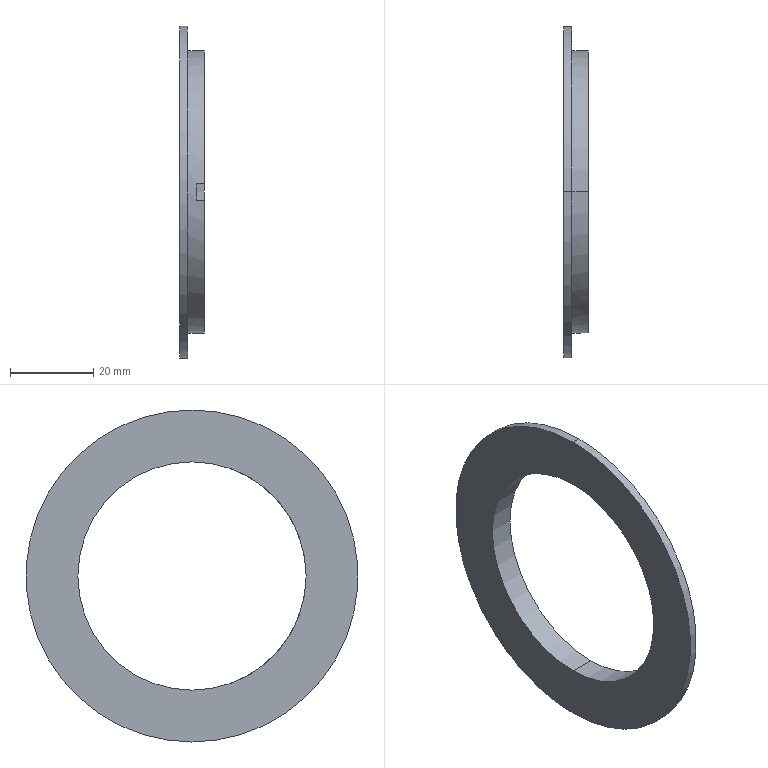Component | SolidWorks | 2InsulatingRing-1 | 1 solid | 12 faces | box 6 x 80 x 80 mm | volume 10273 mm3 | cylinder 6 | plane 6 | commonest cylinder face diameters 55 x2 68 x2 80 x2
build123d program:
from build123d import *

# Parameters (mm, degrees)
SKETCH15_R          = 40
BOSS_EXTRUDE4_DEPTH = 2
SKETCH16_R          = 34
BOSS_EXTRUDE5_DEPTH = 4
SKETCH17_R          = 27.5
CUT_EXTRUDE7_DEPTH  = 34
SKETCH18_W          = 9.008
SKETCH18_H          = 4
CUT_EXTRUDE8_DEPTH  = 57.886


with BuildPart() as part:
    # Sketch15 → Boss-Extrude4 (new body)
    with BuildSketch(Plane(origin=(0, 0, 0), x_dir=(0, 0, -1), z_dir=(1, 0, 0))):
        Circle(SKETCH15_R)
    extrude(amount=BOSS_EXTRUDE4_DEPTH)

    # Sketch16 → Boss-Extrude5 (add)
    with BuildSketch(Plane(origin=(2, 0, 0), x_dir=(0, 0, -1), z_dir=(1, 0, 0))):
        Circle(SKETCH16_R)
    extrude(amount=BOSS_EXTRUDE5_DEPTH)

    # Sketch17 → Cut-Extrude7 (cut)
    with BuildSketch(Plane(origin=(6, 0, 0), x_dir=(0, 0, -1), z_dir=(1, 0, 0))):
        Circle(SKETCH17_R)
    extrude(amount=-CUT_EXTRUDE7_DEPTH, mode=Mode.SUBTRACT)

    # Sketch18 → Cut-Extrude8 (cut, through all)
    with BuildSketch(Plane(origin=(0, 0, 0), x_dir=(1, 0, 0), z_dir=(0, 1, 0))):
        with Locations((8.504, 0)):
            Rectangle(SKETCH18_W, SKETCH18_H)
    extrude(amount=-CUT_EXTRUDE8_DEPTH, mode=Mode.SUBTRACT)


solid = part.part

# Placed as in the assembly
solid = solid.moved(Location((46.957, 1.776, 250), (0, 0, 0)))
STEP:
#1=COLOUR_RGB('',0.7922,0.8196,0.9333);
#2=FILL_AREA_STYLE_COLOUR('',#1);
#3=FILL_AREA_STYLE('',(#2));
#4=SURFACE_STYLE_FILL_AREA(#3);
#5=SURFACE_SIDE_STYLE('',(#4));
#6=SURFACE_STYLE_USAGE(.BOTH.,#5);
#7=PRESENTATION_STYLE_ASSIGNMENT((#6));
#8=CARTESIAN_POINT('',(1.849,0.06992,10.925));
#9=VERTEX_POINT('',#8);
#10=CARTESIAN_POINT('',(1.849,0.06992,8.76));
#11=VERTEX_POINT('',#10);
#12=CARTESIAN_POINT('',(1.849,0.06992,9.843));
#13=DIRECTION('',(1.,0.,0.));
#14=DIRECTION('',(0.,0.,-1.));
#15=AXIS2_PLACEMENT_3D('',#12,#13,#14);
#16=CIRCLE('',#15,1.083);
#17=EDGE_CURVE('',#9,#11,#16,.T.);
#18=ORIENTED_EDGE('',*,*,#17,.F.);
#19=CARTESIAN_POINT('',(2.085,0.06992,10.925));
#20=VERTEX_POINT('',#19);
#21=CARTESIAN_POINT('',(0.7463,0.06992,10.925));
#22=DIRECTION('',(1.,0.,0.));
#23=VECTOR('',#22,39.37);
#24=LINE('',#21,#23);
#25=EDGE_CURVE('',#9,#20,#24,.T.);
#26=ORIENTED_EDGE('',*,*,#25,.T.);
#27=CARTESIAN_POINT('',(2.085,-1.01,9.921));
#28=VERTEX_POINT('',#27);
#29=CARTESIAN_POINT('',(2.085,0.06992,9.843));
#30=DIRECTION('',(1.,0.,0.));
#31=DIRECTION('',(0.,0.,-1.));
#32=AXIS2_PLACEMENT_3D('',#29,#30,#31);
#33=CIRCLE('',#32,1.083);
#34=EDGE_CURVE('',#20,#28,#33,.T.);
#35=ORIENTED_EDGE('',*,*,#34,.T.);
#36=CARTESIAN_POINT('',(2.006,-1.01,9.921));
#37=VERTEX_POINT('',#36);
#38=CARTESIAN_POINT('',(0.7463,-1.01,9.921));
#39=DIRECTION('',(-1.,0.,0.));
#40=VECTOR('',#39,39.37);
#41=LINE('',#38,#40);
#42=EDGE_CURVE('',#28,#37,#41,.T.);
#43=ORIENTED_EDGE('',*,*,#42,.T.);
#44=CARTESIAN_POINT('',(2.006,-1.01,9.764));
#45=VERTEX_POINT('',#44);
#46=CARTESIAN_POINT('',(2.006,0.06992,9.843));
#47=DIRECTION('',(1.,0.,0.));
#48=DIRECTION('',(0.,0.,1.));
#49=AXIS2_PLACEMENT_3D('',#46,#47,#48);
#50=CIRCLE('',#49,1.083);
#51=EDGE_CURVE('',#37,#45,#50,.T.);
#52=ORIENTED_EDGE('',*,*,#51,.T.);
#53=CARTESIAN_POINT('',(2.085,-1.01,9.764));
#54=VERTEX_POINT('',#53);
#55=CARTESIAN_POINT('',(0.7463,-1.01,9.764));
#56=DIRECTION('',(1.,0.,0.));
#57=VECTOR('',#56,39.37);
#58=LINE('',#55,#57);
#59=EDGE_CURVE('',#45,#54,#58,.T.);
#60=ORIENTED_EDGE('',*,*,#59,.T.);
#61=CARTESIAN_POINT('',(2.085,0.06992,8.76));
#62=VERTEX_POINT('',#61);
#63=CARTESIAN_POINT('',(2.085,0.06992,9.843));
#64=DIRECTION('',(1.,0.,0.));
#65=DIRECTION('',(0.,0.,-1.));
#66=AXIS2_PLACEMENT_3D('',#63,#64,#65);
#67=CIRCLE('',#66,1.083);
#68=EDGE_CURVE('',#54,#62,#67,.T.);
#69=ORIENTED_EDGE('',*,*,#68,.T.);
#70=CARTESIAN_POINT('',(0.7463,0.06992,8.76));
#71=DIRECTION('',(1.,0.,0.));
#72=VECTOR('',#71,39.37);
#73=LINE('',#70,#72);
#74=EDGE_CURVE('',#11,#62,#73,.T.);
#75=ORIENTED_EDGE('',*,*,#74,.F.);
#76=EDGE_LOOP('',(#18,#26,#35,#43,#52,#60,#69,#75));
#77=FACE_OUTER_BOUND('',#76,.T.);
#78=CARTESIAN_POINT('',(0.7463,0.06992,9.843));
#79=DIRECTION('',(1.,0.,0.));
#80=DIRECTION('',(0.,0.,-1.));
#81=AXIS2_PLACEMENT_3D('',#78,#79,#80);
#82=CYLINDRICAL_SURFACE('',#81,1.083);
#83=ADVANCED_FACE('',(#77),#82,.F.);
#84=CARTESIAN_POINT('',(2.085,0.06992,8.504));
#85=VERTEX_POINT('',#84);
#86=CARTESIAN_POINT('',(2.085,0.06992,11.181));
#87=VERTEX_POINT('',#86);
#88=CARTESIAN_POINT('',(2.085,0.06992,9.843));
#89=DIRECTION('',(1.,0.,0.));
#90=DIRECTION('',(0.,0.,-1.));
#91=AXIS2_PLACEMENT_3D('',#88,#89,#90);
#92=CIRCLE('',#91,1.339);
#93=EDGE_CURVE('',#85,#87,#92,.T.);
#94=ORIENTED_EDGE('',*,*,#93,.F.);
#95=CARTESIAN_POINT('',(1.927,0.06992,8.504));
#96=VERTEX_POINT('',#95);
#97=CARTESIAN_POINT('',(2.085,0.06992,8.504));
#98=DIRECTION('',(-1.,0.,0.));
#99=VECTOR('',#98,39.37);
#100=LINE('',#97,#99);
#101=EDGE_CURVE('',#85,#96,#100,.T.);
#102=ORIENTED_EDGE('',*,*,#101,.T.);
#103=CARTESIAN_POINT('',(1.927,0.06992,11.181));
#104=VERTEX_POINT('',#103);
#105=CARTESIAN_POINT('',(1.927,0.06992,9.843));
#106=DIRECTION('',(1.,0.,0.));
#107=DIRECTION('',(0.,0.,-1.));
#108=AXIS2_PLACEMENT_3D('',#105,#106,#107);
#109=CIRCLE('',#108,1.339);
#110=EDGE_CURVE('',#96,#104,#109,.T.);
#111=ORIENTED_EDGE('',*,*,#110,.T.);
#112=CARTESIAN_POINT('',(2.085,0.06992,11.181));
#113=DIRECTION('',(-1.,0.,0.));
#114=VECTOR('',#113,39.37);
#115=LINE('',#112,#114);
#116=EDGE_CURVE('',#87,#104,#115,.T.);
#117=ORIENTED_EDGE('',*,*,#116,.F.);
#118=EDGE_LOOP('',(#94,#102,#111,#117));
#119=FACE_OUTER_BOUND('',#118,.T.);
#120=CARTESIAN_POINT('',(2.085,0.06992,9.843));
#121=DIRECTION('',(-1.,0.,0.));
#122=DIRECTION('',(0.,0.,1.));
#123=AXIS2_PLACEMENT_3D('',#120,#121,#122);
#124=CYLINDRICAL_SURFACE('',#123,1.339);
#125=ADVANCED_FACE('',(#119),#124,.T.);
#126=CARTESIAN_POINT('',(1.927,0.06992,8.268));
#127=VERTEX_POINT('',#126);
#128=CARTESIAN_POINT('',(1.927,0.06992,11.417));
#129=VERTEX_POINT('',#128);
#130=CARTESIAN_POINT('',(1.927,0.06992,9.843));
#131=DIRECTION('',(1.,0.,0.));
#132=DIRECTION('',(0.,0.,-1.));
#133=AXIS2_PLACEMENT_3D('',#130,#131,#132);
#134=CIRCLE('',#133,1.575);
#135=EDGE_CURVE('',#127,#129,#134,.T.);
#136=ORIENTED_EDGE('',*,*,#135,.F.);
#137=CARTESIAN_POINT('',(1.849,0.06992,8.268));
#138=VERTEX_POINT('',#137);
#139=CARTESIAN_POINT('',(1.927,0.06992,8.268));
#140=DIRECTION('',(-1.,0.,0.));
#141=VECTOR('',#140,39.37);
#142=LINE('',#139,#141);
#143=EDGE_CURVE('',#127,#138,#142,.T.);
#144=ORIENTED_EDGE('',*,*,#143,.T.);
#145=CARTESIAN_POINT('',(1.849,0.06992,11.417));
#146=VERTEX_POINT('',#145);
#147=CARTESIAN_POINT('',(1.849,0.06992,9.843));
#148=DIRECTION('',(1.,0.,0.));
#149=DIRECTION('',(0.,0.,-1.));
#150=AXIS2_PLACEMENT_3D('',#147,#148,#149);
#151=CIRCLE('',#150,1.575);
#152=EDGE_CURVE('',#138,#146,#151,.T.);
#153=ORIENTED_EDGE('',*,*,#152,.T.);
#154=CARTESIAN_POINT('',(1.927,0.06992,11.417));
#155=DIRECTION('',(-1.,0.,0.));
#156=VECTOR('',#155,39.37);
#157=LINE('',#154,#156);
#158=EDGE_CURVE('',#129,#146,#157,.T.);
#159=ORIENTED_EDGE('',*,*,#158,.F.);
#160=EDGE_LOOP('',(#136,#144,#153,#159));
#161=FACE_OUTER_BOUND('',#160,.T.);
#162=CARTESIAN_POINT('',(1.927,0.06992,9.843));
#163=DIRECTION('',(-1.,0.,0.));
#164=DIRECTION('',(0.,0.,1.));
#165=AXIS2_PLACEMENT_3D('',#162,#163,#164);
#166=CYLINDRICAL_SURFACE('',#165,1.575);
#167=ADVANCED_FACE('',(#161),#166,.T.);
#168=ORIENTED_EDGE('',*,*,#143,.F.);
#169=CARTESIAN_POINT('',(1.927,0.06992,9.843));
#170=DIRECTION('',(1.,0.,0.));
#171=DIRECTION('',(0.,0.,-1.));
#172=AXIS2_PLACEMENT_3D('',#169,#170,#171);
#173=CIRCLE('',#172,1.575);
#174=EDGE_CURVE('',#129,#127,#173,.T.);
#175=ORIENTED_EDGE('',*,*,#174,.F.);
#176=ORIENTED_EDGE('',*,*,#158,.T.);
#177=CARTESIAN_POINT('',(1.849,0.06992,9.843));
#178=DIRECTION('',(1.,0.,0.));
#179=DIRECTION('',(0.,0.,-1.));
#180=AXIS2_PLACEMENT_3D('',#177,#178,#179);
#181=CIRCLE('',#180,1.575);
#182=EDGE_CURVE('',#146,#138,#181,.T.);
#183=ORIENTED_EDGE('',*,*,#182,.T.);
#184=EDGE_LOOP('',(#168,#175,#176,#183));
#185=FACE_OUTER_BOUND('',#184,.T.);
#186=CARTESIAN_POINT('',(1.927,0.06992,9.843));
#187=DIRECTION('',(-1.,0.,0.));
#188=DIRECTION('',(0.,0.,1.));
#189=AXIS2_PLACEMENT_3D('',#186,#187,#188);
#190=CYLINDRICAL_SURFACE('',#189,1.575);
#191=ADVANCED_FACE('',(#185),#190,.T.);
#192=CARTESIAN_POINT('',(1.927,0.06992,9.843));
#193=DIRECTION('',(1.,0.,0.));
#194=DIRECTION('',(0.,0.,-1.));
#195=AXIS2_PLACEMENT_3D('',#192,#193,#194);
#196=CIRCLE('',#195,1.339);
#197=EDGE_CURVE('',#104,#96,#196,.T.);
#198=ORIENTED_EDGE('',*,*,#197,.F.);
#199=ORIENTED_EDGE('',*,*,#110,.F.);
#200=EDGE_LOOP('',(#198,#199));
#201=FACE_BOUND('',#200,.T.);
#202=ORIENTED_EDGE('',*,*,#174,.T.);
#203=ORIENTED_EDGE('',*,*,#135,.T.);
#204=EDGE_LOOP('',(#202,#203));
#205=FACE_OUTER_BOUND('',#204,.T.);
#206=CARTESIAN_POINT('',(1.927,0.06992,9.843));
#207=DIRECTION('',(1.,0.,0.));
#208=DIRECTION('',(0.,0.,-1.));
#209=AXIS2_PLACEMENT_3D('',#206,#207,#208);
#210=PLANE('',#209);
#211=ADVANCED_FACE('',(#201,#205),#210,.T.);
#212=CARTESIAN_POINT('',(1.849,0.06992,9.843));
#213=DIRECTION('',(1.,0.,0.));
#214=DIRECTION('',(0.,0.,-1.));
#215=AXIS2_PLACEMENT_3D('',#212,#213,#214);
#216=CIRCLE('',#215,1.083);
#217=EDGE_CURVE('',#11,#9,#216,.T.);
#218=ORIENTED_EDGE('',*,*,#217,.T.);
#219=ORIENTED_EDGE('',*,*,#17,.T.);
#220=EDGE_LOOP('',(#218,#219));
#221=FACE_BOUND('',#220,.T.);
#222=ORIENTED_EDGE('',*,*,#182,.F.);
#223=ORIENTED_EDGE('',*,*,#152,.F.);
#224=EDGE_LOOP('',(#222,#223));
#225=FACE_OUTER_BOUND('',#224,.T.);
#226=CARTESIAN_POINT('',(1.849,0.06992,9.843));
#227=DIRECTION('',(1.,0.,0.));
#228=DIRECTION('',(0.,0.,-1.));
#229=AXIS2_PLACEMENT_3D('',#226,#227,#228);
#230=PLANE('',#229);
#231=ADVANCED_FACE('',(#221,#225),#230,.F.);
#232=ORIENTED_EDGE('',*,*,#101,.F.);
#233=CARTESIAN_POINT('',(2.085,-1.266,9.764));
#234=VERTEX_POINT('',#233);
#235=CARTESIAN_POINT('',(2.085,0.06992,9.843));
#236=DIRECTION('',(1.,0.,0.));
#237=DIRECTION('',(0.,0.,-1.));
#238=AXIS2_PLACEMENT_3D('',#235,#236,#237);
#239=CIRCLE('',#238,1.339);
#240=EDGE_CURVE('',#234,#85,#239,.T.);
#241=ORIENTED_EDGE('',*,*,#240,.F.);
#242=CARTESIAN_POINT('',(2.006,-1.266,9.764));
#243=VERTEX_POINT('',#242);
#244=CARTESIAN_POINT('',(2.085,-1.266,9.764));
#245=DIRECTION('',(-1.,0.,0.));
#246=VECTOR('',#245,39.37);
#247=LINE('',#244,#246);
#248=EDGE_CURVE('',#234,#243,#247,.T.);
#249=ORIENTED_EDGE('',*,*,#248,.T.);
#250=CARTESIAN_POINT('',(2.006,-1.266,9.921));
#251=VERTEX_POINT('',#250);
#252=CARTESIAN_POINT('',(2.006,0.06992,9.843));
#253=DIRECTION('',(-1.,0.,0.));
#254=DIRECTION('',(0.,0.,1.));
#255=AXIS2_PLACEMENT_3D('',#252,#253,#254);
#256=CIRCLE('',#255,1.339);
#257=EDGE_CURVE('',#243,#251,#256,.T.);
#258=ORIENTED_EDGE('',*,*,#257,.T.);
#259=CARTESIAN_POINT('',(2.085,-1.266,9.921));
#260=VERTEX_POINT('',#259);
#261=CARTESIAN_POINT('',(2.085,-1.266,9.921));
#262=DIRECTION('',(1.,0.,0.));
#263=VECTOR('',#262,39.37);
#264=LINE('',#261,#263);
#265=EDGE_CURVE('',#251,#260,#264,.T.);
#266=ORIENTED_EDGE('',*,*,#265,.T.);
#267=CARTESIAN_POINT('',(2.085,0.06992,9.843));
#268=DIRECTION('',(1.,0.,0.));
#269=DIRECTION('',(0.,0.,-1.));
#270=AXIS2_PLACEMENT_3D('',#267,#268,#269);
#271=CIRCLE('',#270,1.339);
#272=EDGE_CURVE('',#87,#260,#271,.T.);
#273=ORIENTED_EDGE('',*,*,#272,.F.);
#274=ORIENTED_EDGE('',*,*,#116,.T.);
#275=ORIENTED_EDGE('',*,*,#197,.T.);
#276=EDGE_LOOP('',(#232,#241,#249,#258,#266,#273,#274,#275));
#277=FACE_OUTER_BOUND('',#276,.T.);
#278=CARTESIAN_POINT('',(2.085,0.06992,9.843));
#279=DIRECTION('',(-1.,0.,0.));
#280=DIRECTION('',(0.,0.,1.));
#281=AXIS2_PLACEMENT_3D('',#278,#279,#280);
#282=CYLINDRICAL_SURFACE('',#281,1.339);
#283=ADVANCED_FACE('',(#277),#282,.T.);
#284=CARTESIAN_POINT('',(2.085,0.06992,9.764));
#285=DIRECTION('',(0.,1.,0.));
#286=VECTOR('',#285,39.37);
#287=LINE('',#284,#286);
#288=EDGE_CURVE('',#234,#54,#287,.T.);
#289=ORIENTED_EDGE('',*,*,#288,.F.);
#290=ORIENTED_EDGE('',*,*,#240,.T.);
#291=ORIENTED_EDGE('',*,*,#93,.T.);
#292=ORIENTED_EDGE('',*,*,#272,.T.);
#293=CARTESIAN_POINT('',(2.085,0.06992,9.921));
#294=DIRECTION('',(0.,-1.,0.));
#295=VECTOR('',#294,39.37);
#296=LINE('',#293,#295);
#297=EDGE_CURVE('',#28,#260,#296,.T.);
#298=ORIENTED_EDGE('',*,*,#297,.F.);
#299=ORIENTED_EDGE('',*,*,#34,.F.);
#300=CARTESIAN_POINT('',(2.085,0.06992,9.843));
#301=DIRECTION('',(1.,0.,0.));
#302=DIRECTION('',(0.,0.,-1.));
#303=AXIS2_PLACEMENT_3D('',#300,#301,#302);
#304=CIRCLE('',#303,1.083);
#305=EDGE_CURVE('',#62,#20,#304,.T.);
#306=ORIENTED_EDGE('',*,*,#305,.F.);
#307=ORIENTED_EDGE('',*,*,#68,.F.);
#308=EDGE_LOOP('',(#289,#290,#291,#292,#298,#299,#306,#307));
#309=FACE_OUTER_BOUND('',#308,.T.);
#310=CARTESIAN_POINT('',(2.085,0.06992,9.843));
#311=DIRECTION('',(1.,0.,0.));
#312=DIRECTION('',(0.,0.,-1.));
#313=AXIS2_PLACEMENT_3D('',#310,#311,#312);
#314=PLANE('',#313);
#315=ADVANCED_FACE('',(#309),#314,.T.);
#316=ORIENTED_EDGE('',*,*,#25,.F.);
#317=ORIENTED_EDGE('',*,*,#217,.F.);
#318=ORIENTED_EDGE('',*,*,#74,.T.);
#319=ORIENTED_EDGE('',*,*,#305,.T.);
#320=EDGE_LOOP('',(#316,#317,#318,#319));
#321=FACE_OUTER_BOUND('',#320,.T.);
#322=CARTESIAN_POINT('',(0.7463,0.06992,9.843));
#323=DIRECTION('',(1.,0.,0.));
#324=DIRECTION('',(0.,0.,-1.));
#325=AXIS2_PLACEMENT_3D('',#322,#323,#324);
#326=CYLINDRICAL_SURFACE('',#325,1.083);
#327=ADVANCED_FACE('',(#321),#326,.F.);
#328=CARTESIAN_POINT('',(2.006,-1.505,9.764));
#329=DIRECTION('',(0.,1.,0.));
#330=VECTOR('',#329,39.37);
#331=LINE('',#328,#330);
#332=EDGE_CURVE('',#243,#45,#331,.T.);
#333=ORIENTED_EDGE('',*,*,#332,.T.);
#334=ORIENTED_EDGE('',*,*,#51,.F.);
#335=CARTESIAN_POINT('',(2.006,-1.505,9.921));
#336=DIRECTION('',(0.,1.,0.));
#337=VECTOR('',#336,39.37);
#338=LINE('',#335,#337);
#339=EDGE_CURVE('',#251,#37,#338,.T.);
#340=ORIENTED_EDGE('',*,*,#339,.F.);
#341=ORIENTED_EDGE('',*,*,#257,.F.);
#342=EDGE_LOOP('',(#333,#334,#340,#341));
#343=FACE_OUTER_BOUND('',#342,.T.);
#344=CARTESIAN_POINT('',(2.006,-1.505,9.921));
#345=DIRECTION('',(-1.,0.,0.));
#346=DIRECTION('',(0.,0.,1.));
#347=AXIS2_PLACEMENT_3D('',#344,#345,#346);
#348=PLANE('',#347);
#349=ADVANCED_FACE('',(#343),#348,.F.);
#350=ORIENTED_EDGE('',*,*,#288,.T.);
#351=ORIENTED_EDGE('',*,*,#59,.F.);
#352=ORIENTED_EDGE('',*,*,#332,.F.);
#353=ORIENTED_EDGE('',*,*,#248,.F.);
#354=EDGE_LOOP('',(#350,#351,#352,#353));
#355=FACE_OUTER_BOUND('',#354,.T.);
#356=CARTESIAN_POINT('',(2.361,-1.505,9.764));
#357=DIRECTION('',(-0.,0.,-1.));
#358=DIRECTION('',(-1.,0.,0.));
#359=AXIS2_PLACEMENT_3D('',#356,#357,#358);
#360=PLANE('',#359);
#361=ADVANCED_FACE('',(#355),#360,.F.);
#362=ORIENTED_EDGE('',*,*,#339,.T.);
#363=ORIENTED_EDGE('',*,*,#42,.F.);
#364=ORIENTED_EDGE('',*,*,#297,.T.);
#365=ORIENTED_EDGE('',*,*,#265,.F.);
#366=EDGE_LOOP('',(#362,#363,#364,#365));
#367=FACE_OUTER_BOUND('',#366,.T.);
#368=CARTESIAN_POINT('',(2.361,-1.505,9.921));
#369=DIRECTION('',(0.,0.,1.));
#370=DIRECTION('',(1.,0.,-0.));
#371=AXIS2_PLACEMENT_3D('',#368,#369,#370);
#372=PLANE('',#371);
#373=ADVANCED_FACE('',(#367),#372,.F.);
#374=CLOSED_SHELL('',(#83,#125,#167,#191,#211,#231,#283,#315,#327,#349,#361,#373));
#375=MANIFOLD_SOLID_BREP('',#374);
#376=STYLED_ITEM('',(#7),#375);
#377=PRESENTATION_LAYER_ASSIGNMENT('','',(#376));
#378=CARTESIAN_POINT('',(0.,0.,0.));
#379=DIRECTION('',(0.,0.,1.));
#380=DIRECTION('',(1.,0.,0.));
#381=AXIS2_PLACEMENT_3D('',#378,#379,#380);
#382=(LENGTH_UNIT()NAMED_UNIT(*)SI_UNIT($,.METRE.));
#383=LENGTH_MEASURE_WITH_UNIT(LENGTH_MEASURE(0.0254),#382);
#384=DIMENSIONAL_EXPONENTS(1.,0.,0.,0.,0.,0.,0.);
#385=(CONVERSION_BASED_UNIT('',#383)LENGTH_UNIT()NAMED_UNIT(#384));
#386=UNCERTAINTY_MEASURE_WITH_UNIT(LENGTH_MEASURE(0.00001),#385,'','');
#387=(NAMED_UNIT(*)PLANE_ANGLE_UNIT()SI_UNIT($,.RADIAN.));
#388=(NAMED_UNIT(*)SI_UNIT($,.STERADIAN.)SOLID_ANGLE_UNIT());
#389=(GEOMETRIC_REPRESENTATION_CONTEXT(3)GLOBAL_UNCERTAINTY_ASSIGNED_CONTEXT((#386))GLOBAL_UNIT_ASSIGNED_CONTEXT((#385,#387,#388))REPRESENTATION_CONTEXT('',''));
#390=ADVANCED_BREP_SHAPE_REPRESENTATION('',(#375,#381),#389);
#391=(LENGTH_UNIT()NAMED_UNIT(*)SI_UNIT($,.METRE.));
#392=LENGTH_MEASURE_WITH_UNIT(LENGTH_MEASURE(0.0254),#391);
#393=DIMENSIONAL_EXPONENTS(1.,0.,0.,0.,0.,0.,0.);
#394=(CONVERSION_BASED_UNIT('',#392)LENGTH_UNIT()NAMED_UNIT(#393));
#395=UNCERTAINTY_MEASURE_WITH_UNIT(LENGTH_MEASURE(0.00001),#394,'','');
#396=(NAMED_UNIT(*)PLANE_ANGLE_UNIT()SI_UNIT($,.RADIAN.));
#397=(NAMED_UNIT(*)SI_UNIT($,.STERADIAN.)SOLID_ANGLE_UNIT());
#398=(GEOMETRIC_REPRESENTATION_CONTEXT(3)GLOBAL_UNCERTAINTY_ASSIGNED_CONTEXT((#395))GLOBAL_UNIT_ASSIGNED_CONTEXT((#394,#396,#397))REPRESENTATION_CONTEXT('',''));
#399=MECHANICAL_DESIGN_GEOMETRIC_PRESENTATION_REPRESENTATION('',(#376),#398);